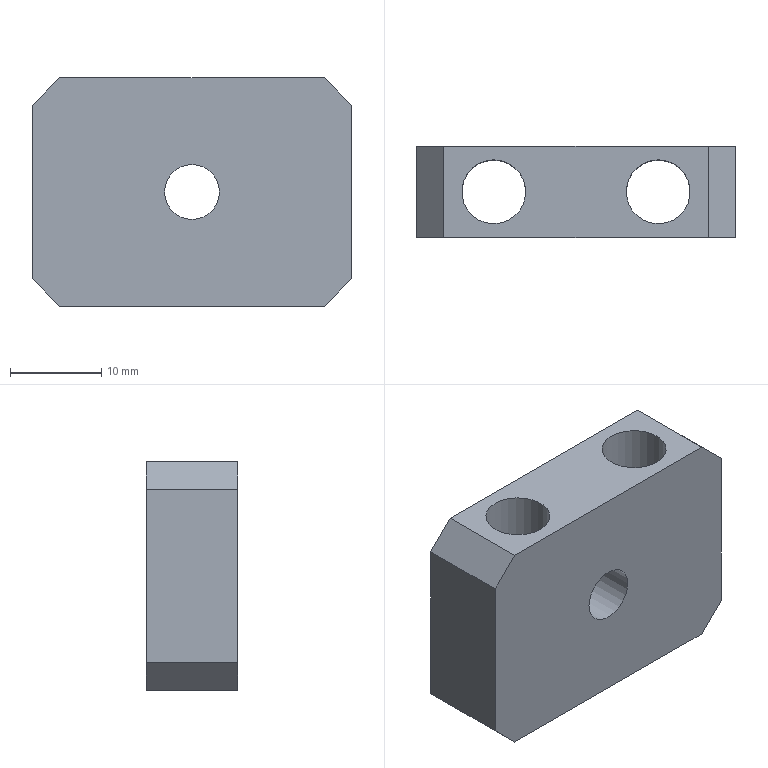Component | NX | CLAMPING_BLOCK | 1 solid | 13 faces | box 35 x 10 x 25 mm | volume 6362 mm3 | plane 10 | cylinder 3 | commonest cylinder face diameters 7 x2 6 x1
STEP:
#1=CARTESIAN_POINT('',(0.,0.,0.));
#2=DIRECTION('',(0.,0.,1.));
#3=DIRECTION('',(1.,0.,0.));
#4=AXIS2_PLACEMENT_3D('',#1,#2,#3);
#5=CARTESIAN_POINT('',(-109.63,80.,105.2));
#6=VERTEX_POINT('',#5);
#7=CARTESIAN_POINT('',(-80.624,80.,105.2));
#8=VERTEX_POINT('',#7);
#9=CARTESIAN_POINT('',(-112.627,80.,105.2));
#10=DIRECTION('',(1.,0.,0.));
#11=VECTOR('',#10,1.);
#12=LINE('',#9,#11);
#13=CARTESIAN_POINT('',(-112.627,80.,105.2));
#14=DIRECTION('',(0.,0.,1.));
#15=DIRECTION('',(0.,-1.,0.));
#16=AXIS2_PLACEMENT_3D('',#13,#14,#15);
#17=PLANE('',#16);
#18=CARTESIAN_POINT('',(0.,0.));
#19=DIRECTION('',(0.,1.));
#20=VECTOR('',#19,1.);
#21=LINE('',#18,#20);
#22=(GEOMETRIC_REPRESENTATION_CONTEXT(2)PARAMETRIC_REPRESENTATION_CONTEXT()REPRESENTATION_CONTEXT('',''));
#23=DEFINITIONAL_REPRESENTATION('',(#21),#22);
#24=PCURVE('',#17,#23);
#25=CARTESIAN_POINT('',(-95.127,80.,117.697));
#26=DIRECTION('',(0.,-1.,0.));
#27=DIRECTION('',(1.,0.,0.));
#28=AXIS2_PLACEMENT_3D('',#25,#26,#27);
#29=PLANE('',#28);
#30=CARTESIAN_POINT('',(-17.5,-12.497));
#31=DIRECTION('',(1.,0.));
#32=VECTOR('',#31,1.);
#33=LINE('',#30,#32);
#34=(GEOMETRIC_REPRESENTATION_CONTEXT(2)PARAMETRIC_REPRESENTATION_CONTEXT()REPRESENTATION_CONTEXT('',''));
#35=DEFINITIONAL_REPRESENTATION('',(#33),#34);
#36=PCURVE('',#29,#35);
#37=SURFACE_CURVE('',#12,(#24,#36),.PCURVE_S1.);
#38=EDGE_CURVE('',#6,#8,#37,.T.);
#39=ORIENTED_EDGE('',*,*,#38,.F.);
#40=CARTESIAN_POINT('',(-109.63,90.,105.2));
#41=VERTEX_POINT('',#40);
#42=CARTESIAN_POINT('',(-109.63,80.,105.2));
#43=DIRECTION('',(0.,1.,0.));
#44=VECTOR('',#43,1.);
#45=LINE('',#42,#44);
#46=CARTESIAN_POINT('',(0.,2.997));
#47=DIRECTION('',(-1.,0.));
#48=VECTOR('',#47,1.);
#49=LINE('',#46,#48);
#50=(GEOMETRIC_REPRESENTATION_CONTEXT(2)PARAMETRIC_REPRESENTATION_CONTEXT()REPRESENTATION_CONTEXT('',''));
#51=DEFINITIONAL_REPRESENTATION('',(#49),#50);
#52=PCURVE('',#17,#51);
#53=CARTESIAN_POINT('',(-109.627,80.,105.197));
#54=DIRECTION('',(0.7071,0.,0.7071));
#55=DIRECTION('',(0.,1.,0.));
#56=AXIS2_PLACEMENT_3D('',#53,#54,#55);
#57=PLANE('',#56);
#58=CARTESIAN_POINT('',(0.,0.004611));
#59=DIRECTION('',(1.,0.));
#60=VECTOR('',#59,1.);
#61=LINE('',#58,#60);
#62=(GEOMETRIC_REPRESENTATION_CONTEXT(2)PARAMETRIC_REPRESENTATION_CONTEXT()REPRESENTATION_CONTEXT('',''));
#63=DEFINITIONAL_REPRESENTATION('',(#61),#62);
#64=PCURVE('',#57,#63);
#65=SURFACE_CURVE('',#45,(#52,#64),.PCURVE_S1.);
#66=EDGE_CURVE('',#6,#41,#65,.T.);
#67=ORIENTED_EDGE('',*,*,#66,.T.);
#68=CARTESIAN_POINT('',(-80.624,90.,105.2));
#69=VERTEX_POINT('',#68);
#70=CARTESIAN_POINT('',(-112.627,90.,105.2));
#71=DIRECTION('',(1.,0.,0.));
#72=VECTOR('',#71,1.);
#73=LINE('',#70,#72);
#74=CARTESIAN_POINT('',(-10.,0.));
#75=DIRECTION('',(0.,1.));
#76=VECTOR('',#75,1.);
#77=LINE('',#74,#76);
#78=(GEOMETRIC_REPRESENTATION_CONTEXT(2)PARAMETRIC_REPRESENTATION_CONTEXT()REPRESENTATION_CONTEXT('',''));
#79=DEFINITIONAL_REPRESENTATION('',(#77),#78);
#80=PCURVE('',#17,#79);
#81=CARTESIAN_POINT('',(-95.127,90.,117.697));
#82=DIRECTION('',(0.,-1.,0.));
#83=DIRECTION('',(1.,0.,0.));
#84=AXIS2_PLACEMENT_3D('',#81,#82,#83);
#85=PLANE('',#84);
#86=CARTESIAN_POINT('',(-17.5,-12.497));
#87=DIRECTION('',(1.,0.));
#88=VECTOR('',#87,1.);
#89=LINE('',#86,#88);
#90=(GEOMETRIC_REPRESENTATION_CONTEXT(2)PARAMETRIC_REPRESENTATION_CONTEXT()REPRESENTATION_CONTEXT('',''));
#91=DEFINITIONAL_REPRESENTATION('',(#89),#90);
#92=PCURVE('',#85,#91);
#93=SURFACE_CURVE('',#73,(#80,#92),.PCURVE_S1.);
#94=EDGE_CURVE('',#41,#69,#93,.T.);
#95=ORIENTED_EDGE('',*,*,#94,.T.);
#96=CARTESIAN_POINT('',(-80.624,80.,105.2));
#97=DIRECTION('',(0.,-1.,0.));
#98=VECTOR('',#97,1.);
#99=LINE('',#96,#98);
#100=CARTESIAN_POINT('',(0.,32.003));
#101=DIRECTION('',(1.,0.));
#102=VECTOR('',#101,1.);
#103=LINE('',#100,#102);
#104=(GEOMETRIC_REPRESENTATION_CONTEXT(2)PARAMETRIC_REPRESENTATION_CONTEXT()REPRESENTATION_CONTEXT('',''));
#105=DEFINITIONAL_REPRESENTATION('',(#103),#104);
#106=PCURVE('',#17,#105);
#107=CARTESIAN_POINT('',(-77.627,80.,108.197));
#108=DIRECTION('',(-0.7071,0.,0.7071));
#109=DIRECTION('',(0.,1.,0.));
#110=AXIS2_PLACEMENT_3D('',#107,#108,#109);
#111=PLANE('',#110);
#112=CARTESIAN_POINT('',(0.,4.238));
#113=DIRECTION('',(-1.,0.));
#114=VECTOR('',#113,1.);
#115=LINE('',#112,#114);
#116=(GEOMETRIC_REPRESENTATION_CONTEXT(2)PARAMETRIC_REPRESENTATION_CONTEXT()REPRESENTATION_CONTEXT('',''));
#117=DEFINITIONAL_REPRESENTATION('',(#115),#116);
#118=PCURVE('',#111,#117);
#119=SURFACE_CURVE('',#99,(#106,#118),.PCURVE_S1.);
#120=EDGE_CURVE('',#69,#8,#119,.T.);
#121=ORIENTED_EDGE('',*,*,#120,.T.);
#122=EDGE_LOOP('',(#39,#67,#95,#121));
#123=FACE_BOUND('',#122,.T.);
#124=CARTESIAN_POINT('',(-104.127,81.5,105.2));
#125=VERTEX_POINT('',#124);
#126=CARTESIAN_POINT('',(-104.127,85.,105.2));
#127=DIRECTION('',(0.,0.,-1.));
#128=DIRECTION('',(0.,-1.,0.));
#129=AXIS2_PLACEMENT_3D('',#126,#127,#128);
#130=CIRCLE('',#129,3.5);
#131=CARTESIAN_POINT('',(-1.5,8.5));
#132=CARTESIAN_POINT('',(-1.5,2.438));
#133=CARTESIAN_POINT('',(-6.75,5.469));
#134=CARTESIAN_POINT('',(-12.,8.5));
#135=CARTESIAN_POINT('',(-6.75,11.531));
#136=CARTESIAN_POINT('',(-1.5,14.562));
#137=CARTESIAN_POINT('',(-1.5,8.5));
#138=(BOUNDED_CURVE()B_SPLINE_CURVE(2,(#131,#132,#133,#134,#135,#136,#137),.UNSPECIFIED.,.T.,.F.)B_SPLINE_CURVE_WITH_KNOTS((1,2,2,2,2,1),(-2.094,0.,2.094,4.189,6.283,8.378),.UNSPECIFIED.)CURVE()GEOMETRIC_REPRESENTATION_ITEM()RATIONAL_B_SPLINE_CURVE((1.,0.5,1.,0.5,1.,0.5,1.))REPRESENTATION_ITEM(''));
#139=(GEOMETRIC_REPRESENTATION_CONTEXT(2)PARAMETRIC_REPRESENTATION_CONTEXT()REPRESENTATION_CONTEXT('',''));
#140=DEFINITIONAL_REPRESENTATION('',(#138),#139);
#141=PCURVE('',#17,#140);
#142=CARTESIAN_POINT('',(-104.127,85.,97.697));
#143=DIRECTION('',(0.,0.,1.));
#144=DIRECTION('',(0.,-1.,0.));
#145=AXIS2_PLACEMENT_3D('',#142,#143,#144);
#146=CYLINDRICAL_SURFACE('',#145,3.5);
#147=CARTESIAN_POINT('',(6.283,7.503));
#148=DIRECTION('',(-1.,0.));
#149=VECTOR('',#148,1.);
#150=LINE('',#147,#149);
#151=(GEOMETRIC_REPRESENTATION_CONTEXT(2)PARAMETRIC_REPRESENTATION_CONTEXT()REPRESENTATION_CONTEXT('',''));
#152=DEFINITIONAL_REPRESENTATION('',(#150),#151);
#153=PCURVE('',#146,#152);
#154=SURFACE_CURVE('',#130,(#141,#153),.PCURVE_S1.);
#155=EDGE_CURVE('',#125,#125,#154,.T.);
#156=ORIENTED_EDGE('',*,*,#155,.F.);
#157=EDGE_LOOP('',(#156));
#158=FACE_BOUND('',#157,.T.);
#159=CARTESIAN_POINT('',(-86.127,81.5,105.2));
#160=VERTEX_POINT('',#159);
#161=CARTESIAN_POINT('',(-86.127,85.,105.2));
#162=DIRECTION('',(0.,0.,1.));
#163=DIRECTION('',(0.,-1.,0.));
#164=AXIS2_PLACEMENT_3D('',#161,#162,#163);
#165=CIRCLE('',#164,3.5);
#166=CARTESIAN_POINT('',(-5.,26.5));
#167=DIRECTION('',(1.,0.));
#168=AXIS2_PLACEMENT_2D('',#166,#167);
#169=CIRCLE('',#168,3.5);
#170=(GEOMETRIC_REPRESENTATION_CONTEXT(2)PARAMETRIC_REPRESENTATION_CONTEXT()REPRESENTATION_CONTEXT('',''));
#171=DEFINITIONAL_REPRESENTATION('',(#169),#170);
#172=PCURVE('',#17,#171);
#173=CARTESIAN_POINT('',(-86.127,85.,97.697));
#174=DIRECTION('',(0.,0.,1.));
#175=DIRECTION('',(0.,-1.,0.));
#176=AXIS2_PLACEMENT_3D('',#173,#174,#175);
#177=CYLINDRICAL_SURFACE('',#176,3.5);
#178=CARTESIAN_POINT('',(0.,7.503));
#179=DIRECTION('',(1.,0.));
#180=VECTOR('',#179,1.);
#181=LINE('',#178,#180);
#182=(GEOMETRIC_REPRESENTATION_CONTEXT(2)PARAMETRIC_REPRESENTATION_CONTEXT()REPRESENTATION_CONTEXT('',''));
#183=DEFINITIONAL_REPRESENTATION('',(#181),#182);
#184=PCURVE('',#177,#183);
#185=SURFACE_CURVE('',#165,(#172,#184),.PCURVE_S1.);
#186=EDGE_CURVE('',#160,#160,#185,.T.);
#187=ORIENTED_EDGE('',*,*,#186,.T.);
#188=EDGE_LOOP('',(#187));
#189=FACE_BOUND('',#188,.T.);
#190=ADVANCED_FACE('',(#123,#158,#189),#17,.F.);
#191=CARTESIAN_POINT('',(-80.627,90.,130.197));
#192=VERTEX_POINT('',#191);
#193=CARTESIAN_POINT('',(-109.627,90.,130.197));
#194=VERTEX_POINT('',#193);
#195=CARTESIAN_POINT('',(-77.627,90.,130.197));
#196=DIRECTION('',(-1.,0.,0.));
#197=VECTOR('',#196,1.);
#198=LINE('',#195,#197);
#199=CARTESIAN_POINT('',(-77.627,80.,130.197));
#200=DIRECTION('',(0.,0.,-1.));
#201=DIRECTION('',(0.,1.,0.));
#202=AXIS2_PLACEMENT_3D('',#199,#200,#201);
#203=PLANE('',#202);
#204=CARTESIAN_POINT('',(10.,0.));
#205=DIRECTION('',(0.,-1.));
#206=VECTOR('',#205,1.);
#207=LINE('',#204,#206);
#208=(GEOMETRIC_REPRESENTATION_CONTEXT(2)PARAMETRIC_REPRESENTATION_CONTEXT()REPRESENTATION_CONTEXT('',''));
#209=DEFINITIONAL_REPRESENTATION('',(#207),#208);
#210=PCURVE('',#203,#209);
#211=CARTESIAN_POINT('',(17.5,12.5));
#212=DIRECTION('',(-1.,0.));
#213=VECTOR('',#212,1.);
#214=LINE('',#211,#213);
#215=(GEOMETRIC_REPRESENTATION_CONTEXT(2)PARAMETRIC_REPRESENTATION_CONTEXT()REPRESENTATION_CONTEXT('',''));
#216=DEFINITIONAL_REPRESENTATION('',(#214),#215);
#217=PCURVE('',#85,#216);
#218=SURFACE_CURVE('',#198,(#210,#217),.PCURVE_S1.);
#219=EDGE_CURVE('',#192,#194,#218,.T.);
#220=ORIENTED_EDGE('',*,*,#219,.T.);
#221=CARTESIAN_POINT('',(-109.627,80.,130.197));
#222=VERTEX_POINT('',#221);
#223=CARTESIAN_POINT('',(-109.627,80.,130.197));
#224=DIRECTION('',(0.,-1.,0.));
#225=VECTOR('',#224,1.);
#226=LINE('',#223,#225);
#227=CARTESIAN_POINT('',(0.,-32.));
#228=DIRECTION('',(-1.,0.));
#229=VECTOR('',#228,1.);
#230=LINE('',#227,#229);
#231=(GEOMETRIC_REPRESENTATION_CONTEXT(2)PARAMETRIC_REPRESENTATION_CONTEXT()REPRESENTATION_CONTEXT('',''));
#232=DEFINITIONAL_REPRESENTATION('',(#230),#231);
#233=PCURVE('',#203,#232);
#234=CARTESIAN_POINT('',(-112.627,80.,127.197));
#235=DIRECTION('',(0.7071,0.,-0.7071));
#236=DIRECTION('',(0.,1.,0.));
#237=AXIS2_PLACEMENT_3D('',#234,#235,#236);
#238=PLANE('',#237);
#239=CARTESIAN_POINT('',(0.,4.243));
#240=DIRECTION('',(-1.,0.));
#241=VECTOR('',#240,1.);
#242=LINE('',#239,#241);
#243=(GEOMETRIC_REPRESENTATION_CONTEXT(2)PARAMETRIC_REPRESENTATION_CONTEXT()REPRESENTATION_CONTEXT('',''));
#244=DEFINITIONAL_REPRESENTATION('',(#242),#243);
#245=PCURVE('',#238,#244);
#246=SURFACE_CURVE('',#226,(#233,#245),.PCURVE_S1.);
#247=EDGE_CURVE('',#194,#222,#246,.T.);
#248=ORIENTED_EDGE('',*,*,#247,.T.);
#249=CARTESIAN_POINT('',(-80.627,80.,130.197));
#250=VERTEX_POINT('',#249);
#251=CARTESIAN_POINT('',(-77.627,80.,130.197));
#252=DIRECTION('',(-1.,0.,0.));
#253=VECTOR('',#252,1.);
#254=LINE('',#251,#253);
#255=CARTESIAN_POINT('',(0.,0.));
#256=DIRECTION('',(0.,-1.));
#257=VECTOR('',#256,1.);
#258=LINE('',#255,#257);
#259=(GEOMETRIC_REPRESENTATION_CONTEXT(2)PARAMETRIC_REPRESENTATION_CONTEXT()REPRESENTATION_CONTEXT('',''));
#260=DEFINITIONAL_REPRESENTATION('',(#258),#259);
#261=PCURVE('',#203,#260);
#262=CARTESIAN_POINT('',(17.5,12.5));
#263=DIRECTION('',(-1.,0.));
#264=VECTOR('',#263,1.);
#265=LINE('',#262,#264);
#266=(GEOMETRIC_REPRESENTATION_CONTEXT(2)PARAMETRIC_REPRESENTATION_CONTEXT()REPRESENTATION_CONTEXT('',''));
#267=DEFINITIONAL_REPRESENTATION('',(#265),#266);
#268=PCURVE('',#29,#267);
#269=SURFACE_CURVE('',#254,(#261,#268),.PCURVE_S1.);
#270=EDGE_CURVE('',#250,#222,#269,.T.);
#271=ORIENTED_EDGE('',*,*,#270,.F.);
#272=CARTESIAN_POINT('',(-80.627,80.,130.197));
#273=DIRECTION('',(0.,1.,0.));
#274=VECTOR('',#273,1.);
#275=LINE('',#272,#274);
#276=CARTESIAN_POINT('',(0.,-3.));
#277=DIRECTION('',(1.,0.));
#278=VECTOR('',#277,1.);
#279=LINE('',#276,#278);
#280=(GEOMETRIC_REPRESENTATION_CONTEXT(2)PARAMETRIC_REPRESENTATION_CONTEXT()REPRESENTATION_CONTEXT('',''));
#281=DEFINITIONAL_REPRESENTATION('',(#279),#280);
#282=PCURVE('',#203,#281);
#283=CARTESIAN_POINT('',(-80.627,80.,130.197));
#284=DIRECTION('',(-0.7071,0.,-0.7071));
#285=DIRECTION('',(0.,1.,0.));
#286=AXIS2_PLACEMENT_3D('',#283,#284,#285);
#287=PLANE('',#286);
#288=CARTESIAN_POINT('',(0.,0.));
#289=DIRECTION('',(1.,0.));
#290=VECTOR('',#289,1.);
#291=LINE('',#288,#290);
#292=(GEOMETRIC_REPRESENTATION_CONTEXT(2)PARAMETRIC_REPRESENTATION_CONTEXT()REPRESENTATION_CONTEXT('',''));
#293=DEFINITIONAL_REPRESENTATION('',(#291),#292);
#294=PCURVE('',#287,#293);
#295=SURFACE_CURVE('',#275,(#282,#294),.PCURVE_S1.);
#296=EDGE_CURVE('',#250,#192,#295,.T.);
#297=ORIENTED_EDGE('',*,*,#296,.T.);
#298=EDGE_LOOP('',(#220,#248,#271,#297));
#299=FACE_BOUND('',#298,.T.);
#300=CARTESIAN_POINT('',(-104.127,88.5,130.197));
#301=VERTEX_POINT('',#300);
#302=CARTESIAN_POINT('',(-104.127,81.5,130.197));
#303=VERTEX_POINT('',#302);
#304=CARTESIAN_POINT('',(-104.127,85.,130.197));
#305=DIRECTION('',(0.,0.,1.));
#306=DIRECTION('',(0.,1.,0.));
#307=AXIS2_PLACEMENT_3D('',#304,#305,#306);
#308=CIRCLE('',#307,3.5);
#309=CARTESIAN_POINT('',(8.5,-26.5));
#310=CARTESIAN_POINT('',(8.5,-32.562));
#311=CARTESIAN_POINT('',(3.25,-29.531));
#312=CARTESIAN_POINT('',(-2.,-26.5));
#313=CARTESIAN_POINT('',(3.25,-23.469));
#314=CARTESIAN_POINT('',(8.5,-20.438));
#315=CARTESIAN_POINT('',(8.5,-26.5));
#316=(BOUNDED_CURVE()B_SPLINE_CURVE(2,(#309,#310,#311,#312,#313,#314,#315),.UNSPECIFIED.,.T.,.F.)B_SPLINE_CURVE_WITH_KNOTS((1,2,2,2,2,1),(-2.094,0.,2.094,4.189,6.283,8.378),.UNSPECIFIED.)CURVE()GEOMETRIC_REPRESENTATION_ITEM()RATIONAL_B_SPLINE_CURVE((1.,0.5,1.,0.5,1.,0.5,1.))REPRESENTATION_ITEM(''));
#317=(GEOMETRIC_REPRESENTATION_CONTEXT(2)PARAMETRIC_REPRESENTATION_CONTEXT()REPRESENTATION_CONTEXT('',''));
#318=DEFINITIONAL_REPRESENTATION('',(#316),#317);
#319=PCURVE('',#203,#318);
#320=CARTESIAN_POINT('',(3.142,32.5));
#321=DIRECTION('',(1.,0.));
#322=VECTOR('',#321,1.);
#323=LINE('',#320,#322);
#324=(GEOMETRIC_REPRESENTATION_CONTEXT(2)PARAMETRIC_REPRESENTATION_CONTEXT()REPRESENTATION_CONTEXT('',''));
#325=DEFINITIONAL_REPRESENTATION('',(#323),#324);
#326=PCURVE('',#146,#325);
#327=SURFACE_CURVE('',#308,(#319,#326),.PCURVE_S1.);
#328=EDGE_CURVE('',#301,#303,#327,.T.);
#329=ORIENTED_EDGE('',*,*,#328,.F.);
#330=CARTESIAN_POINT('',(-104.127,85.,130.197));
#331=DIRECTION('',(0.,0.,1.));
#332=DIRECTION('',(0.,1.,0.));
#333=AXIS2_PLACEMENT_3D('',#330,#331,#332);
#334=CIRCLE('',#333,3.5);
#335=CARTESIAN_POINT('',(8.5,-26.5));
#336=CARTESIAN_POINT('',(8.5,-32.562));
#337=CARTESIAN_POINT('',(3.25,-29.531));
#338=CARTESIAN_POINT('',(-2.,-26.5));
#339=CARTESIAN_POINT('',(3.25,-23.469));
#340=CARTESIAN_POINT('',(8.5,-20.438));
#341=CARTESIAN_POINT('',(8.5,-26.5));
#342=(BOUNDED_CURVE()B_SPLINE_CURVE(2,(#335,#336,#337,#338,#339,#340,#341),.UNSPECIFIED.,.T.,.F.)B_SPLINE_CURVE_WITH_KNOTS((1,2,2,2,2,1),(-2.094,0.,2.094,4.189,6.283,8.378),.UNSPECIFIED.)CURVE()GEOMETRIC_REPRESENTATION_ITEM()RATIONAL_B_SPLINE_CURVE((1.,0.5,1.,0.5,1.,0.5,1.))REPRESENTATION_ITEM(''));
#343=(GEOMETRIC_REPRESENTATION_CONTEXT(2)PARAMETRIC_REPRESENTATION_CONTEXT()REPRESENTATION_CONTEXT('',''));
#344=DEFINITIONAL_REPRESENTATION('',(#342),#343);
#345=PCURVE('',#203,#344);
#346=CARTESIAN_POINT('',(-3.142,32.5));
#347=DIRECTION('',(1.,0.));
#348=VECTOR('',#347,1.);
#349=LINE('',#346,#348);
#350=(GEOMETRIC_REPRESENTATION_CONTEXT(2)PARAMETRIC_REPRESENTATION_CONTEXT()REPRESENTATION_CONTEXT('',''));
#351=DEFINITIONAL_REPRESENTATION('',(#349),#350);
#352=PCURVE('',#146,#351);
#353=SURFACE_CURVE('',#334,(#345,#352),.PCURVE_S1.);
#354=EDGE_CURVE('',#303,#301,#353,.T.);
#355=ORIENTED_EDGE('',*,*,#354,.F.);
#356=EDGE_LOOP('',(#329,#355));
#357=FACE_BOUND('',#356,.T.);
#358=CARTESIAN_POINT('',(-86.127,88.5,130.197));
#359=VERTEX_POINT('',#358);
#360=CARTESIAN_POINT('',(-86.127,81.5,130.197));
#361=VERTEX_POINT('',#360);
#362=CARTESIAN_POINT('',(-86.127,85.,130.197));
#363=DIRECTION('',(0.,0.,-1.));
#364=DIRECTION('',(0.,1.,0.));
#365=AXIS2_PLACEMENT_3D('',#362,#363,#364);
#366=CIRCLE('',#365,3.5);
#367=CARTESIAN_POINT('',(5.,-8.5));
#368=DIRECTION('',(1.,0.));
#369=AXIS2_PLACEMENT_2D('',#367,#368);
#370=CIRCLE('',#369,3.5);
#371=(GEOMETRIC_REPRESENTATION_CONTEXT(2)PARAMETRIC_REPRESENTATION_CONTEXT()REPRESENTATION_CONTEXT('',''));
#372=DEFINITIONAL_REPRESENTATION('',(#370),#371);
#373=PCURVE('',#203,#372);
#374=CARTESIAN_POINT('',(3.142,32.5));
#375=DIRECTION('',(-1.,0.));
#376=VECTOR('',#375,1.);
#377=LINE('',#374,#376);
#378=(GEOMETRIC_REPRESENTATION_CONTEXT(2)PARAMETRIC_REPRESENTATION_CONTEXT()REPRESENTATION_CONTEXT('',''));
#379=DEFINITIONAL_REPRESENTATION('',(#377),#378);
#380=PCURVE('',#177,#379);
#381=SURFACE_CURVE('',#366,(#373,#380),.PCURVE_S1.);
#382=EDGE_CURVE('',#359,#361,#381,.T.);
#383=ORIENTED_EDGE('',*,*,#382,.T.);
#384=CARTESIAN_POINT('',(-86.127,85.,130.197));
#385=DIRECTION('',(0.,0.,-1.));
#386=DIRECTION('',(0.,1.,0.));
#387=AXIS2_PLACEMENT_3D('',#384,#385,#386);
#388=CIRCLE('',#387,3.5);
#389=CARTESIAN_POINT('',(5.,-8.5));
#390=DIRECTION('',(1.,0.));
#391=AXIS2_PLACEMENT_2D('',#389,#390);
#392=CIRCLE('',#391,3.5);
#393=(GEOMETRIC_REPRESENTATION_CONTEXT(2)PARAMETRIC_REPRESENTATION_CONTEXT()REPRESENTATION_CONTEXT('',''));
#394=DEFINITIONAL_REPRESENTATION('',(#392),#393);
#395=PCURVE('',#203,#394);
#396=CARTESIAN_POINT('',(9.425,32.5));
#397=DIRECTION('',(-1.,0.));
#398=VECTOR('',#397,1.);
#399=LINE('',#396,#398);
#400=(GEOMETRIC_REPRESENTATION_CONTEXT(2)PARAMETRIC_REPRESENTATION_CONTEXT()REPRESENTATION_CONTEXT('',''));
#401=DEFINITIONAL_REPRESENTATION('',(#399),#400);
#402=PCURVE('',#177,#401);
#403=SURFACE_CURVE('',#388,(#395,#402),.PCURVE_S1.);
#404=EDGE_CURVE('',#361,#359,#403,.T.);
#405=ORIENTED_EDGE('',*,*,#404,.T.);
#406=EDGE_LOOP('',(#383,#405));
#407=FACE_BOUND('',#406,.T.);
#408=ADVANCED_FACE('',(#299,#357,#407),#203,.F.);
#409=CARTESIAN_POINT('',(-112.627,80.,127.197));
#410=VERTEX_POINT('',#409);
#411=CARTESIAN_POINT('',(-112.627,80.,108.197));
#412=VERTEX_POINT('',#411);
#413=CARTESIAN_POINT('',(-112.627,80.,130.197));
#414=DIRECTION('',(0.,0.,-1.));
#415=VECTOR('',#414,1.);
#416=LINE('',#413,#415);
#417=CARTESIAN_POINT('',(-112.627,80.,130.197));
#418=DIRECTION('',(1.,0.,0.));
#419=DIRECTION('',(0.,1.,0.));
#420=AXIS2_PLACEMENT_3D('',#417,#418,#419);
#421=PLANE('',#420);
#422=CARTESIAN_POINT('',(0.,0.));
#423=DIRECTION('',(0.,-1.));
#424=VECTOR('',#423,1.);
#425=LINE('',#422,#424);
#426=(GEOMETRIC_REPRESENTATION_CONTEXT(2)PARAMETRIC_REPRESENTATION_CONTEXT()REPRESENTATION_CONTEXT('',''));
#427=DEFINITIONAL_REPRESENTATION('',(#425),#426);
#428=PCURVE('',#421,#427);
#429=CARTESIAN_POINT('',(-17.5,12.5));
#430=DIRECTION('',(0.,-1.));
#431=VECTOR('',#430,1.);
#432=LINE('',#429,#431);
#433=(GEOMETRIC_REPRESENTATION_CONTEXT(2)PARAMETRIC_REPRESENTATION_CONTEXT()REPRESENTATION_CONTEXT('',''));
#434=DEFINITIONAL_REPRESENTATION('',(#432),#433);
#435=PCURVE('',#29,#434);
#436=SURFACE_CURVE('',#416,(#428,#435),.PCURVE_S1.);
#437=EDGE_CURVE('',#410,#412,#436,.T.);
#438=ORIENTED_EDGE('',*,*,#437,.F.);
#439=CARTESIAN_POINT('',(-112.627,90.,127.197));
#440=VERTEX_POINT('',#439);
#441=CARTESIAN_POINT('',(-112.627,80.,127.197));
#442=DIRECTION('',(0.,1.,0.));
#443=VECTOR('',#442,1.);
#444=LINE('',#441,#443);
#445=CARTESIAN_POINT('',(0.,-3.));
#446=DIRECTION('',(1.,0.));
#447=VECTOR('',#446,1.);
#448=LINE('',#445,#447);
#449=(GEOMETRIC_REPRESENTATION_CONTEXT(2)PARAMETRIC_REPRESENTATION_CONTEXT()REPRESENTATION_CONTEXT('',''));
#450=DEFINITIONAL_REPRESENTATION('',(#448),#449);
#451=PCURVE('',#421,#450);
#452=CARTESIAN_POINT('',(0.,0.));
#453=DIRECTION('',(1.,0.));
#454=VECTOR('',#453,1.);
#455=LINE('',#452,#454);
#456=(GEOMETRIC_REPRESENTATION_CONTEXT(2)PARAMETRIC_REPRESENTATION_CONTEXT()REPRESENTATION_CONTEXT('',''));
#457=DEFINITIONAL_REPRESENTATION('',(#455),#456);
#458=PCURVE('',#238,#457);
#459=SURFACE_CURVE('',#444,(#451,#458),.PCURVE_S1.);
#460=EDGE_CURVE('',#410,#440,#459,.T.);
#461=ORIENTED_EDGE('',*,*,#460,.T.);
#462=CARTESIAN_POINT('',(-112.627,90.,108.197));
#463=VERTEX_POINT('',#462);
#464=CARTESIAN_POINT('',(-112.627,90.,130.197));
#465=DIRECTION('',(0.,0.,-1.));
#466=VECTOR('',#465,1.);
#467=LINE('',#464,#466);
#468=CARTESIAN_POINT('',(10.,0.));
#469=DIRECTION('',(0.,-1.));
#470=VECTOR('',#469,1.);
#471=LINE('',#468,#470);
#472=(GEOMETRIC_REPRESENTATION_CONTEXT(2)PARAMETRIC_REPRESENTATION_CONTEXT()REPRESENTATION_CONTEXT('',''));
#473=DEFINITIONAL_REPRESENTATION('',(#471),#472);
#474=PCURVE('',#421,#473);
#475=CARTESIAN_POINT('',(-17.5,12.5));
#476=DIRECTION('',(0.,-1.));
#477=VECTOR('',#476,1.);
#478=LINE('',#475,#477);
#479=(GEOMETRIC_REPRESENTATION_CONTEXT(2)PARAMETRIC_REPRESENTATION_CONTEXT()REPRESENTATION_CONTEXT('',''));
#480=DEFINITIONAL_REPRESENTATION('',(#478),#479);
#481=PCURVE('',#85,#480);
#482=SURFACE_CURVE('',#467,(#474,#481),.PCURVE_S1.);
#483=EDGE_CURVE('',#440,#463,#482,.T.);
#484=ORIENTED_EDGE('',*,*,#483,.T.);
#485=CARTESIAN_POINT('',(-112.627,80.,108.197));
#486=DIRECTION('',(0.,-1.,0.));
#487=VECTOR('',#486,1.);
#488=LINE('',#485,#487);
#489=CARTESIAN_POINT('',(0.,-22.));
#490=DIRECTION('',(-1.,0.));
#491=VECTOR('',#490,1.);
#492=LINE('',#489,#491);
#493=(GEOMETRIC_REPRESENTATION_CONTEXT(2)PARAMETRIC_REPRESENTATION_CONTEXT()REPRESENTATION_CONTEXT('',''));
#494=DEFINITIONAL_REPRESENTATION('',(#492),#493);
#495=PCURVE('',#421,#494);
#496=CARTESIAN_POINT('',(0.,4.243));
#497=DIRECTION('',(-1.,0.));
#498=VECTOR('',#497,1.);
#499=LINE('',#496,#498);
#500=(GEOMETRIC_REPRESENTATION_CONTEXT(2)PARAMETRIC_REPRESENTATION_CONTEXT()REPRESENTATION_CONTEXT('',''));
#501=DEFINITIONAL_REPRESENTATION('',(#499),#500);
#502=PCURVE('',#57,#501);
#503=SURFACE_CURVE('',#488,(#495,#502),.PCURVE_S1.);
#504=EDGE_CURVE('',#463,#412,#503,.T.);
#505=ORIENTED_EDGE('',*,*,#504,.T.);
#506=EDGE_LOOP('',(#438,#461,#484,#505));
#507=FACE_BOUND('',#506,.T.);
#508=ADVANCED_FACE('',(#507),#421,.F.);
#509=CARTESIAN_POINT('',(-77.627,90.,108.197));
#510=VERTEX_POINT('',#509);
#511=CARTESIAN_POINT('',(-77.627,90.,127.197));
#512=VERTEX_POINT('',#511);
#513=CARTESIAN_POINT('',(-77.627,90.,105.197));
#514=DIRECTION('',(0.,0.,1.));
#515=VECTOR('',#514,1.);
#516=LINE('',#513,#515);
#517=CARTESIAN_POINT('',(-77.627,80.,105.197));
#518=DIRECTION('',(-1.,0.,0.));
#519=DIRECTION('',(0.,-1.,0.));
#520=AXIS2_PLACEMENT_3D('',#517,#518,#519);
#521=PLANE('',#520);
#522=CARTESIAN_POINT('',(-10.,0.));
#523=DIRECTION('',(0.,1.));
#524=VECTOR('',#523,1.);
#525=LINE('',#522,#524);
#526=(GEOMETRIC_REPRESENTATION_CONTEXT(2)PARAMETRIC_REPRESENTATION_CONTEXT()REPRESENTATION_CONTEXT('',''));
#527=DEFINITIONAL_REPRESENTATION('',(#525),#526);
#528=PCURVE('',#521,#527);
#529=CARTESIAN_POINT('',(17.5,-12.5));
#530=DIRECTION('',(0.,1.));
#531=VECTOR('',#530,1.);
#532=LINE('',#529,#531);
#533=(GEOMETRIC_REPRESENTATION_CONTEXT(2)PARAMETRIC_REPRESENTATION_CONTEXT()REPRESENTATION_CONTEXT('',''));
#534=DEFINITIONAL_REPRESENTATION('',(#532),#533);
#535=PCURVE('',#85,#534);
#536=SURFACE_CURVE('',#516,(#528,#535),.PCURVE_S1.);
#537=EDGE_CURVE('',#510,#512,#536,.T.);
#538=ORIENTED_EDGE('',*,*,#537,.T.);
#539=CARTESIAN_POINT('',(-77.627,80.,127.197));
#540=VERTEX_POINT('',#539);
#541=CARTESIAN_POINT('',(-77.627,80.,127.197));
#542=DIRECTION('',(0.,-1.,0.));
#543=VECTOR('',#542,1.);
#544=LINE('',#541,#543);
#545=CARTESIAN_POINT('',(0.,22.));
#546=DIRECTION('',(1.,0.));
#547=VECTOR('',#546,1.);
#548=LINE('',#545,#547);
#549=(GEOMETRIC_REPRESENTATION_CONTEXT(2)PARAMETRIC_REPRESENTATION_CONTEXT()REPRESENTATION_CONTEXT('',''));
#550=DEFINITIONAL_REPRESENTATION('',(#548),#549);
#551=PCURVE('',#521,#550);
#552=CARTESIAN_POINT('',(0.,4.243));
#553=DIRECTION('',(-1.,0.));
#554=VECTOR('',#553,1.);
#555=LINE('',#552,#554);
#556=(GEOMETRIC_REPRESENTATION_CONTEXT(2)PARAMETRIC_REPRESENTATION_CONTEXT()REPRESENTATION_CONTEXT('',''));
#557=DEFINITIONAL_REPRESENTATION('',(#555),#556);
#558=PCURVE('',#287,#557);
#559=SURFACE_CURVE('',#544,(#551,#558),.PCURVE_S1.);
#560=EDGE_CURVE('',#512,#540,#559,.T.);
#561=ORIENTED_EDGE('',*,*,#560,.T.);
#562=CARTESIAN_POINT('',(-77.627,80.,108.197));
#563=VERTEX_POINT('',#562);
#564=CARTESIAN_POINT('',(-77.627,80.,105.197));
#565=DIRECTION('',(0.,0.,1.));
#566=VECTOR('',#565,1.);
#567=LINE('',#564,#566);
#568=CARTESIAN_POINT('',(0.,0.));
#569=DIRECTION('',(0.,1.));
#570=VECTOR('',#569,1.);
#571=LINE('',#568,#570);
#572=(GEOMETRIC_REPRESENTATION_CONTEXT(2)PARAMETRIC_REPRESENTATION_CONTEXT()REPRESENTATION_CONTEXT('',''));
#573=DEFINITIONAL_REPRESENTATION('',(#571),#572);
#574=PCURVE('',#521,#573);
#575=CARTESIAN_POINT('',(17.5,-12.5));
#576=DIRECTION('',(0.,1.));
#577=VECTOR('',#576,1.);
#578=LINE('',#575,#577);
#579=(GEOMETRIC_REPRESENTATION_CONTEXT(2)PARAMETRIC_REPRESENTATION_CONTEXT()REPRESENTATION_CONTEXT('',''));
#580=DEFINITIONAL_REPRESENTATION('',(#578),#579);
#581=PCURVE('',#29,#580);
#582=SURFACE_CURVE('',#567,(#574,#581),.PCURVE_S1.);
#583=EDGE_CURVE('',#563,#540,#582,.T.);
#584=ORIENTED_EDGE('',*,*,#583,.F.);
#585=CARTESIAN_POINT('',(-77.627,80.,108.197));
#586=DIRECTION('',(0.,1.,0.));
#587=VECTOR('',#586,1.);
#588=LINE('',#585,#587);
#589=CARTESIAN_POINT('',(0.,3.));
#590=DIRECTION('',(-1.,0.));
#591=VECTOR('',#590,1.);
#592=LINE('',#589,#591);
#593=(GEOMETRIC_REPRESENTATION_CONTEXT(2)PARAMETRIC_REPRESENTATION_CONTEXT()REPRESENTATION_CONTEXT('',''));
#594=DEFINITIONAL_REPRESENTATION('',(#592),#593);
#595=PCURVE('',#521,#594);
#596=CARTESIAN_POINT('',(0.,0.));
#597=DIRECTION('',(1.,0.));
#598=VECTOR('',#597,1.);
#599=LINE('',#596,#598);
#600=(GEOMETRIC_REPRESENTATION_CONTEXT(2)PARAMETRIC_REPRESENTATION_CONTEXT()REPRESENTATION_CONTEXT('',''));
#601=DEFINITIONAL_REPRESENTATION('',(#599),#600);
#602=PCURVE('',#111,#601);
#603=SURFACE_CURVE('',#588,(#595,#602),.PCURVE_S1.);
#604=EDGE_CURVE('',#563,#510,#603,.T.);
#605=ORIENTED_EDGE('',*,*,#604,.T.);
#606=EDGE_LOOP('',(#538,#561,#584,#605));
#607=FACE_BOUND('',#606,.T.);
#608=ADVANCED_FACE('',(#607),#521,.F.);
#609=CARTESIAN_POINT('',(-92.127,80.,117.697));
#610=VERTEX_POINT('',#609);
#611=CARTESIAN_POINT('',(-95.127,80.,117.697));
#612=DIRECTION('',(0.,1.,0.));
#613=DIRECTION('',(1.,0.,0.));
#614=AXIS2_PLACEMENT_3D('',#611,#612,#613);
#615=CIRCLE('',#614,3.);
#616=CARTESIAN_POINT('',(3.,0.));
#617=CARTESIAN_POINT('',(3.,-5.196));
#618=CARTESIAN_POINT('',(-1.5,-2.598));
#619=CARTESIAN_POINT('',(-6.,-0.));
#620=CARTESIAN_POINT('',(-1.5,2.598));
#621=CARTESIAN_POINT('',(3.,5.196));
#622=CARTESIAN_POINT('',(3.,0.));
#623=(BOUNDED_CURVE()B_SPLINE_CURVE(2,(#616,#617,#618,#619,#620,#621,#622),.UNSPECIFIED.,.T.,.F.)B_SPLINE_CURVE_WITH_KNOTS((1,2,2,2,2,1),(-2.094,0.,2.094,4.189,6.283,8.378),.UNSPECIFIED.)CURVE()GEOMETRIC_REPRESENTATION_ITEM()RATIONAL_B_SPLINE_CURVE((1.,0.5,1.,0.5,1.,0.5,1.))REPRESENTATION_ITEM(''));
#624=(GEOMETRIC_REPRESENTATION_CONTEXT(2)PARAMETRIC_REPRESENTATION_CONTEXT()REPRESENTATION_CONTEXT('',''));
#625=DEFINITIONAL_REPRESENTATION('',(#623),#624);
#626=PCURVE('',#29,#625);
#627=CARTESIAN_POINT('',(-95.127,120.,117.697));
#628=DIRECTION('',(0.,-1.,0.));
#629=DIRECTION('',(1.,0.,0.));
#630=AXIS2_PLACEMENT_3D('',#627,#628,#629);
#631=CYLINDRICAL_SURFACE('',#630,3.);
#632=CARTESIAN_POINT('',(6.283,40.));
#633=DIRECTION('',(-1.,0.));
#634=VECTOR('',#633,1.);
#635=LINE('',#632,#634);
#636=(GEOMETRIC_REPRESENTATION_CONTEXT(2)PARAMETRIC_REPRESENTATION_CONTEXT()REPRESENTATION_CONTEXT('',''));
#637=DEFINITIONAL_REPRESENTATION('',(#635),#636);
#638=PCURVE('',#631,#637);
#639=SURFACE_CURVE('',#615,(#626,#638),.PCURVE_S1.);
#640=EDGE_CURVE('',#610,#610,#639,.T.);
#641=ORIENTED_EDGE('',*,*,#640,.T.);
#642=EDGE_LOOP('',(#641));
#643=FACE_BOUND('',#642,.T.);
#644=ORIENTED_EDGE('',*,*,#270,.T.);
#645=CARTESIAN_POINT('',(-108.627,80.,131.197));
#646=DIRECTION('',(-0.7071,0.,-0.7071));
#647=VECTOR('',#646,1.);
#648=LINE('',#645,#647);
#649=CARTESIAN_POINT('',(-13.5,13.5));
#650=DIRECTION('',(-0.7071,-0.7071));
#651=VECTOR('',#650,1.);
#652=LINE('',#649,#651);
#653=(GEOMETRIC_REPRESENTATION_CONTEXT(2)PARAMETRIC_REPRESENTATION_CONTEXT()REPRESENTATION_CONTEXT('',''));
#654=DEFINITIONAL_REPRESENTATION('',(#652),#653);
#655=PCURVE('',#29,#654);
#656=CARTESIAN_POINT('',(0.,5.657));
#657=DIRECTION('',(0.,-1.));
#658=VECTOR('',#657,1.);
#659=LINE('',#656,#658);
#660=(GEOMETRIC_REPRESENTATION_CONTEXT(2)PARAMETRIC_REPRESENTATION_CONTEXT()REPRESENTATION_CONTEXT('',''));
#661=DEFINITIONAL_REPRESENTATION('',(#659),#660);
#662=PCURVE('',#238,#661);
#663=SURFACE_CURVE('',#648,(#655,#662),.PCURVE_S1.);
#664=EDGE_CURVE('',#222,#410,#663,.T.);
#665=ORIENTED_EDGE('',*,*,#664,.T.);
#666=ORIENTED_EDGE('',*,*,#437,.T.);
#667=CARTESIAN_POINT('',(-108.627,80.,104.197));
#668=DIRECTION('',(0.7071,0.,-0.7071));
#669=VECTOR('',#668,1.);
#670=LINE('',#667,#669);
#671=CARTESIAN_POINT('',(-13.5,-13.5));
#672=DIRECTION('',(0.7071,-0.7071));
#673=VECTOR('',#672,1.);
#674=LINE('',#671,#673);
#675=(GEOMETRIC_REPRESENTATION_CONTEXT(2)PARAMETRIC_REPRESENTATION_CONTEXT()REPRESENTATION_CONTEXT('',''));
#676=DEFINITIONAL_REPRESENTATION('',(#674),#675);
#677=PCURVE('',#29,#676);
#678=CARTESIAN_POINT('',(0.,-1.414));
#679=DIRECTION('',(0.,-1.));
#680=VECTOR('',#679,1.);
#681=LINE('',#678,#680);
#682=(GEOMETRIC_REPRESENTATION_CONTEXT(2)PARAMETRIC_REPRESENTATION_CONTEXT()REPRESENTATION_CONTEXT('',''));
#683=DEFINITIONAL_REPRESENTATION('',(#681),#682);
#684=PCURVE('',#57,#683);
#685=SURFACE_CURVE('',#670,(#677,#684),.PCURVE_S1.);
#686=EDGE_CURVE('',#412,#6,#685,.T.);
#687=ORIENTED_EDGE('',*,*,#686,.T.);
#688=ORIENTED_EDGE('',*,*,#38,.T.);
#689=CARTESIAN_POINT('',(-81.627,80.,104.197));
#690=DIRECTION('',(0.7071,0.,0.7071));
#691=VECTOR('',#690,1.);
#692=LINE('',#689,#691);
#693=CARTESIAN_POINT('',(13.5,-13.5));
#694=DIRECTION('',(0.7071,0.7071));
#695=VECTOR('',#694,1.);
#696=LINE('',#693,#695);
#697=(GEOMETRIC_REPRESENTATION_CONTEXT(2)PARAMETRIC_REPRESENTATION_CONTEXT()REPRESENTATION_CONTEXT('',''));
#698=DEFINITIONAL_REPRESENTATION('',(#696),#697);
#699=PCURVE('',#29,#698);
#700=CARTESIAN_POINT('',(0.,5.657));
#701=DIRECTION('',(0.,-1.));
#702=VECTOR('',#701,1.);
#703=LINE('',#700,#702);
#704=(GEOMETRIC_REPRESENTATION_CONTEXT(2)PARAMETRIC_REPRESENTATION_CONTEXT()REPRESENTATION_CONTEXT('',''));
#705=DEFINITIONAL_REPRESENTATION('',(#703),#704);
#706=PCURVE('',#111,#705);
#707=SURFACE_CURVE('',#692,(#699,#706),.PCURVE_S1.);
#708=EDGE_CURVE('',#8,#563,#707,.T.);
#709=ORIENTED_EDGE('',*,*,#708,.T.);
#710=ORIENTED_EDGE('',*,*,#583,.T.);
#711=CARTESIAN_POINT('',(-81.627,80.,131.197));
#712=DIRECTION('',(-0.7071,0.,0.7071));
#713=VECTOR('',#712,1.);
#714=LINE('',#711,#713);
#715=CARTESIAN_POINT('',(13.5,13.5));
#716=DIRECTION('',(-0.7071,0.7071));
#717=VECTOR('',#716,1.);
#718=LINE('',#715,#717);
#719=(GEOMETRIC_REPRESENTATION_CONTEXT(2)PARAMETRIC_REPRESENTATION_CONTEXT()REPRESENTATION_CONTEXT('',''));
#720=DEFINITIONAL_REPRESENTATION('',(#718),#719);
#721=PCURVE('',#29,#720);
#722=CARTESIAN_POINT('',(0.,-1.414));
#723=DIRECTION('',(0.,-1.));
#724=VECTOR('',#723,1.);
#725=LINE('',#722,#724);
#726=(GEOMETRIC_REPRESENTATION_CONTEXT(2)PARAMETRIC_REPRESENTATION_CONTEXT()REPRESENTATION_CONTEXT('',''));
#727=DEFINITIONAL_REPRESENTATION('',(#725),#726);
#728=PCURVE('',#287,#727);
#729=SURFACE_CURVE('',#714,(#721,#728),.PCURVE_S1.);
#730=EDGE_CURVE('',#540,#250,#729,.T.);
#731=ORIENTED_EDGE('',*,*,#730,.T.);
#732=EDGE_LOOP('',(#644,#665,#666,#687,#688,#709,#710,#731));
#733=FACE_BOUND('',#732,.T.);
#734=ADVANCED_FACE('',(#643,#733),#29,.T.);
#735=CARTESIAN_POINT('',(-92.127,90.,117.697));
#736=VERTEX_POINT('',#735);
#737=CARTESIAN_POINT('',(-95.127,90.,117.697));
#738=DIRECTION('',(0.,1.,0.));
#739=DIRECTION('',(1.,0.,0.));
#740=AXIS2_PLACEMENT_3D('',#737,#738,#739);
#741=CIRCLE('',#740,3.);
#742=CARTESIAN_POINT('',(3.,0.));
#743=CARTESIAN_POINT('',(3.,-5.196));
#744=CARTESIAN_POINT('',(-1.5,-2.598));
#745=CARTESIAN_POINT('',(-6.,-0.));
#746=CARTESIAN_POINT('',(-1.5,2.598));
#747=CARTESIAN_POINT('',(3.,5.196));
#748=CARTESIAN_POINT('',(3.,0.));
#749=(BOUNDED_CURVE()B_SPLINE_CURVE(2,(#742,#743,#744,#745,#746,#747,#748),.UNSPECIFIED.,.T.,.F.)B_SPLINE_CURVE_WITH_KNOTS((1,2,2,2,2,1),(-2.094,0.,2.094,4.189,6.283,8.378),.UNSPECIFIED.)CURVE()GEOMETRIC_REPRESENTATION_ITEM()RATIONAL_B_SPLINE_CURVE((1.,0.5,1.,0.5,1.,0.5,1.))REPRESENTATION_ITEM(''));
#750=(GEOMETRIC_REPRESENTATION_CONTEXT(2)PARAMETRIC_REPRESENTATION_CONTEXT()REPRESENTATION_CONTEXT('',''));
#751=DEFINITIONAL_REPRESENTATION('',(#749),#750);
#752=PCURVE('',#85,#751);
#753=CARTESIAN_POINT('',(6.283,30.));
#754=DIRECTION('',(-1.,0.));
#755=VECTOR('',#754,1.);
#756=LINE('',#753,#755);
#757=(GEOMETRIC_REPRESENTATION_CONTEXT(2)PARAMETRIC_REPRESENTATION_CONTEXT()REPRESENTATION_CONTEXT('',''));
#758=DEFINITIONAL_REPRESENTATION('',(#756),#757);
#759=PCURVE('',#631,#758);
#760=SURFACE_CURVE('',#741,(#752,#759),.PCURVE_S1.);
#761=EDGE_CURVE('',#736,#736,#760,.T.);
#762=ORIENTED_EDGE('',*,*,#761,.F.);
#763=EDGE_LOOP('',(#762));
#764=FACE_BOUND('',#763,.T.);
#765=ORIENTED_EDGE('',*,*,#483,.F.);
#766=CARTESIAN_POINT('',(-112.627,90.,127.197));
#767=DIRECTION('',(0.7071,0.,0.7071));
#768=VECTOR('',#767,1.);
#769=LINE('',#766,#768);
#770=CARTESIAN_POINT('',(-17.5,9.5));
#771=DIRECTION('',(0.7071,0.7071));
#772=VECTOR('',#771,1.);
#773=LINE('',#770,#772);
#774=(GEOMETRIC_REPRESENTATION_CONTEXT(2)PARAMETRIC_REPRESENTATION_CONTEXT()REPRESENTATION_CONTEXT('',''));
#775=DEFINITIONAL_REPRESENTATION('',(#773),#774);
#776=PCURVE('',#85,#775);
#777=CARTESIAN_POINT('',(10.,0.));
#778=DIRECTION('',(0.,1.));
#779=VECTOR('',#778,1.);
#780=LINE('',#777,#779);
#781=(GEOMETRIC_REPRESENTATION_CONTEXT(2)PARAMETRIC_REPRESENTATION_CONTEXT()REPRESENTATION_CONTEXT('',''));
#782=DEFINITIONAL_REPRESENTATION('',(#780),#781);
#783=PCURVE('',#238,#782);
#784=SURFACE_CURVE('',#769,(#776,#783),.PCURVE_S1.);
#785=EDGE_CURVE('',#440,#194,#784,.T.);
#786=ORIENTED_EDGE('',*,*,#785,.T.);
#787=ORIENTED_EDGE('',*,*,#219,.F.);
#788=CARTESIAN_POINT('',(-80.627,90.,130.197));
#789=DIRECTION('',(0.7071,0.,-0.7071));
#790=VECTOR('',#789,1.);
#791=LINE('',#788,#790);
#792=CARTESIAN_POINT('',(14.5,12.5));
#793=DIRECTION('',(0.7071,-0.7071));
#794=VECTOR('',#793,1.);
#795=LINE('',#792,#794);
#796=(GEOMETRIC_REPRESENTATION_CONTEXT(2)PARAMETRIC_REPRESENTATION_CONTEXT()REPRESENTATION_CONTEXT('',''));
#797=DEFINITIONAL_REPRESENTATION('',(#795),#796);
#798=PCURVE('',#85,#797);
#799=CARTESIAN_POINT('',(10.,0.));
#800=DIRECTION('',(0.,1.));
#801=VECTOR('',#800,1.);
#802=LINE('',#799,#801);
#803=(GEOMETRIC_REPRESENTATION_CONTEXT(2)PARAMETRIC_REPRESENTATION_CONTEXT()REPRESENTATION_CONTEXT('',''));
#804=DEFINITIONAL_REPRESENTATION('',(#802),#803);
#805=PCURVE('',#287,#804);
#806=SURFACE_CURVE('',#791,(#798,#805),.PCURVE_S1.);
#807=EDGE_CURVE('',#192,#512,#806,.T.);
#808=ORIENTED_EDGE('',*,*,#807,.T.);
#809=ORIENTED_EDGE('',*,*,#537,.F.);
#810=CARTESIAN_POINT('',(-77.627,90.,108.197));
#811=DIRECTION('',(-0.7071,0.,-0.7071));
#812=VECTOR('',#811,1.);
#813=LINE('',#810,#812);
#814=CARTESIAN_POINT('',(17.5,-9.5));
#815=DIRECTION('',(-0.7071,-0.7071));
#816=VECTOR('',#815,1.);
#817=LINE('',#814,#816);
#818=(GEOMETRIC_REPRESENTATION_CONTEXT(2)PARAMETRIC_REPRESENTATION_CONTEXT()REPRESENTATION_CONTEXT('',''));
#819=DEFINITIONAL_REPRESENTATION('',(#817),#818);
#820=PCURVE('',#85,#819);
#821=CARTESIAN_POINT('',(10.,0.));
#822=DIRECTION('',(0.,1.));
#823=VECTOR('',#822,1.);
#824=LINE('',#821,#823);
#825=(GEOMETRIC_REPRESENTATION_CONTEXT(2)PARAMETRIC_REPRESENTATION_CONTEXT()REPRESENTATION_CONTEXT('',''));
#826=DEFINITIONAL_REPRESENTATION('',(#824),#825);
#827=PCURVE('',#111,#826);
#828=SURFACE_CURVE('',#813,(#820,#827),.PCURVE_S1.);
#829=EDGE_CURVE('',#510,#69,#828,.T.);
#830=ORIENTED_EDGE('',*,*,#829,.T.);
#831=ORIENTED_EDGE('',*,*,#94,.F.);
#832=CARTESIAN_POINT('',(-109.627,90.,105.197));
#833=DIRECTION('',(-0.7071,0.,0.7071));
#834=VECTOR('',#833,1.);
#835=LINE('',#832,#834);
#836=CARTESIAN_POINT('',(-14.5,-12.5));
#837=DIRECTION('',(-0.7071,0.7071));
#838=VECTOR('',#837,1.);
#839=LINE('',#836,#838);
#840=(GEOMETRIC_REPRESENTATION_CONTEXT(2)PARAMETRIC_REPRESENTATION_CONTEXT()REPRESENTATION_CONTEXT('',''));
#841=DEFINITIONAL_REPRESENTATION('',(#839),#840);
#842=PCURVE('',#85,#841);
#843=CARTESIAN_POINT('',(10.,0.));
#844=DIRECTION('',(0.,1.));
#845=VECTOR('',#844,1.);
#846=LINE('',#843,#845);
#847=(GEOMETRIC_REPRESENTATION_CONTEXT(2)PARAMETRIC_REPRESENTATION_CONTEXT()REPRESENTATION_CONTEXT('',''));
#848=DEFINITIONAL_REPRESENTATION('',(#846),#847);
#849=PCURVE('',#57,#848);
#850=SURFACE_CURVE('',#835,(#842,#849),.PCURVE_S1.);
#851=EDGE_CURVE('',#41,#463,#850,.T.);
#852=ORIENTED_EDGE('',*,*,#851,.T.);
#853=EDGE_LOOP('',(#765,#786,#787,#808,#809,#830,#831,#852));
#854=FACE_BOUND('',#853,.T.);
#855=ADVANCED_FACE('',(#764,#854),#85,.F.);
#856=ORIENTED_EDGE('',*,*,#664,.F.);
#857=ORIENTED_EDGE('',*,*,#247,.F.);
#858=ORIENTED_EDGE('',*,*,#785,.F.);
#859=ORIENTED_EDGE('',*,*,#460,.F.);
#860=EDGE_LOOP('',(#856,#857,#858,#859));
#861=FACE_BOUND('',#860,.T.);
#862=ADVANCED_FACE('',(#861),#238,.F.);
#863=ORIENTED_EDGE('',*,*,#686,.F.);
#864=ORIENTED_EDGE('',*,*,#504,.F.);
#865=ORIENTED_EDGE('',*,*,#851,.F.);
#866=ORIENTED_EDGE('',*,*,#66,.F.);
#867=EDGE_LOOP('',(#863,#864,#865,#866));
#868=FACE_BOUND('',#867,.T.);
#869=ADVANCED_FACE('',(#868),#57,.F.);
#870=ORIENTED_EDGE('',*,*,#730,.F.);
#871=ORIENTED_EDGE('',*,*,#560,.F.);
#872=ORIENTED_EDGE('',*,*,#807,.F.);
#873=ORIENTED_EDGE('',*,*,#296,.F.);
#874=EDGE_LOOP('',(#870,#871,#872,#873));
#875=FACE_BOUND('',#874,.T.);
#876=ADVANCED_FACE('',(#875),#287,.F.);
#877=ORIENTED_EDGE('',*,*,#708,.F.);
#878=ORIENTED_EDGE('',*,*,#120,.F.);
#879=ORIENTED_EDGE('',*,*,#829,.F.);
#880=ORIENTED_EDGE('',*,*,#604,.F.);
#881=EDGE_LOOP('',(#877,#878,#879,#880));
#882=FACE_BOUND('',#881,.T.);
#883=ADVANCED_FACE('',(#882),#111,.F.);
#884=ORIENTED_EDGE('',*,*,#354,.F.);
#885=CARTESIAN_POINT('',(-104.127,81.5,105.2));
#886=CARTESIAN_POINT('',(-104.127,81.5,130.197));
#887=B_SPLINE_CURVE_WITH_KNOTS('',1,(#885,#886),.UNSPECIFIED.,.F.,.F.,(2,2),(7.503,32.5),.PIECEWISE_BEZIER_KNOTS.);
#888=CARTESIAN_POINT('',(0.,0.));
#889=DIRECTION('',(0.,1.));
#890=VECTOR('',#889,1.);
#891=LINE('',#888,#890);
#892=(GEOMETRIC_REPRESENTATION_CONTEXT(2)PARAMETRIC_REPRESENTATION_CONTEXT()REPRESENTATION_CONTEXT('',''));
#893=DEFINITIONAL_REPRESENTATION('',(#891),#892);
#894=PCURVE('',#146,#893);
#895=CARTESIAN_POINT('',(6.283,0.));
#896=DIRECTION('',(0.,1.));
#897=VECTOR('',#896,1.);
#898=LINE('',#895,#897);
#899=(GEOMETRIC_REPRESENTATION_CONTEXT(2)PARAMETRIC_REPRESENTATION_CONTEXT()REPRESENTATION_CONTEXT('',''));
#900=DEFINITIONAL_REPRESENTATION('',(#898),#899);
#901=PCURVE('',#146,#900);
#902=SEAM_CURVE('',#887,(#894,#901),.PCURVE_S1.);
#903=EDGE_CURVE('',#125,#303,#902,.T.);
#904=ORIENTED_EDGE('',*,*,#903,.F.);
#905=ORIENTED_EDGE('',*,*,#155,.F.);
#906=ORIENTED_EDGE('',*,*,#903,.T.);
#907=ORIENTED_EDGE('',*,*,#328,.F.);
#908=EDGE_LOOP('',(#884,#904,#905,#906,#907));
#909=FACE_BOUND('',#908,.F.);
#910=ADVANCED_FACE('',(#909),#146,.F.);
#911=ORIENTED_EDGE('',*,*,#382,.T.);
#912=CARTESIAN_POINT('',(-86.127,81.5,105.2));
#913=CARTESIAN_POINT('',(-86.127,81.5,130.197));
#914=B_SPLINE_CURVE_WITH_KNOTS('',1,(#912,#913),.UNSPECIFIED.,.F.,.F.,(2,2),(7.503,32.5),.PIECEWISE_BEZIER_KNOTS.);
#915=CARTESIAN_POINT('',(0.,0.));
#916=DIRECTION('',(0.,1.));
#917=VECTOR('',#916,1.);
#918=LINE('',#915,#917);
#919=(GEOMETRIC_REPRESENTATION_CONTEXT(2)PARAMETRIC_REPRESENTATION_CONTEXT()REPRESENTATION_CONTEXT('',''));
#920=DEFINITIONAL_REPRESENTATION('',(#918),#919);
#921=PCURVE('',#177,#920);
#922=CARTESIAN_POINT('',(6.283,0.));
#923=DIRECTION('',(0.,1.));
#924=VECTOR('',#923,1.);
#925=LINE('',#922,#924);
#926=(GEOMETRIC_REPRESENTATION_CONTEXT(2)PARAMETRIC_REPRESENTATION_CONTEXT()REPRESENTATION_CONTEXT('',''));
#927=DEFINITIONAL_REPRESENTATION('',(#925),#926);
#928=PCURVE('',#177,#927);
#929=SEAM_CURVE('',#914,(#921,#928),.PCURVE_S1.);
#930=EDGE_CURVE('',#160,#361,#929,.T.);
#931=ORIENTED_EDGE('',*,*,#930,.F.);
#932=ORIENTED_EDGE('',*,*,#186,.T.);
#933=ORIENTED_EDGE('',*,*,#930,.T.);
#934=ORIENTED_EDGE('',*,*,#404,.T.);
#935=EDGE_LOOP('',(#911,#931,#932,#933,#934));
#936=FACE_BOUND('',#935,.F.);
#937=ADVANCED_FACE('',(#936),#177,.F.);
#938=ORIENTED_EDGE('',*,*,#640,.T.);
#939=CARTESIAN_POINT('',(-92.127,90.,117.697));
#940=CARTESIAN_POINT('',(-92.127,80.,117.697));
#941=B_SPLINE_CURVE_WITH_KNOTS('',1,(#939,#940),.UNSPECIFIED.,.F.,.F.,(2,2),(30.,40.),.PIECEWISE_BEZIER_KNOTS.);
#942=CARTESIAN_POINT('',(0.,0.));
#943=DIRECTION('',(0.,1.));
#944=VECTOR('',#943,1.);
#945=LINE('',#942,#944);
#946=(GEOMETRIC_REPRESENTATION_CONTEXT(2)PARAMETRIC_REPRESENTATION_CONTEXT()REPRESENTATION_CONTEXT('',''));
#947=DEFINITIONAL_REPRESENTATION('',(#945),#946);
#948=PCURVE('',#631,#947);
#949=CARTESIAN_POINT('',(6.283,0.));
#950=DIRECTION('',(0.,1.));
#951=VECTOR('',#950,1.);
#952=LINE('',#949,#951);
#953=(GEOMETRIC_REPRESENTATION_CONTEXT(2)PARAMETRIC_REPRESENTATION_CONTEXT()REPRESENTATION_CONTEXT('',''));
#954=DEFINITIONAL_REPRESENTATION('',(#952),#953);
#955=PCURVE('',#631,#954);
#956=SEAM_CURVE('',#941,(#948,#955),.PCURVE_S1.);
#957=EDGE_CURVE('',#736,#610,#956,.T.);
#958=ORIENTED_EDGE('',*,*,#957,.F.);
#959=ORIENTED_EDGE('',*,*,#761,.F.);
#960=ORIENTED_EDGE('',*,*,#957,.T.);
#961=EDGE_LOOP('',(#938,#958,#959,#960));
#962=FACE_BOUND('',#961,.F.);
#963=ADVANCED_FACE('',(#962),#631,.F.);
#964=CLOSED_SHELL('',(#190,#408,#508,#608,#734,#855,#862,#869,#876,#883,#910,#937,#963));
#965=MANIFOLD_SOLID_BREP('',#964);
#966=(LENGTH_UNIT()NAMED_UNIT(*)SI_UNIT(.MILLI.,.METRE.));
#967=UNCERTAINTY_MEASURE_WITH_UNIT(LENGTH_MEASURE(0.000002),#966,'','');
#968=(NAMED_UNIT(*)PLANE_ANGLE_UNIT()SI_UNIT($,.RADIAN.));
#969=(NAMED_UNIT(*)SI_UNIT($,.STERADIAN.)SOLID_ANGLE_UNIT());
#970=(GEOMETRIC_REPRESENTATION_CONTEXT(3)GLOBAL_UNCERTAINTY_ASSIGNED_CONTEXT((#967))GLOBAL_UNIT_ASSIGNED_CONTEXT((#966,#968,#969))REPRESENTATION_CONTEXT('',''));
#971=ADVANCED_BREP_SHAPE_REPRESENTATION('',(#4,#965),#970);